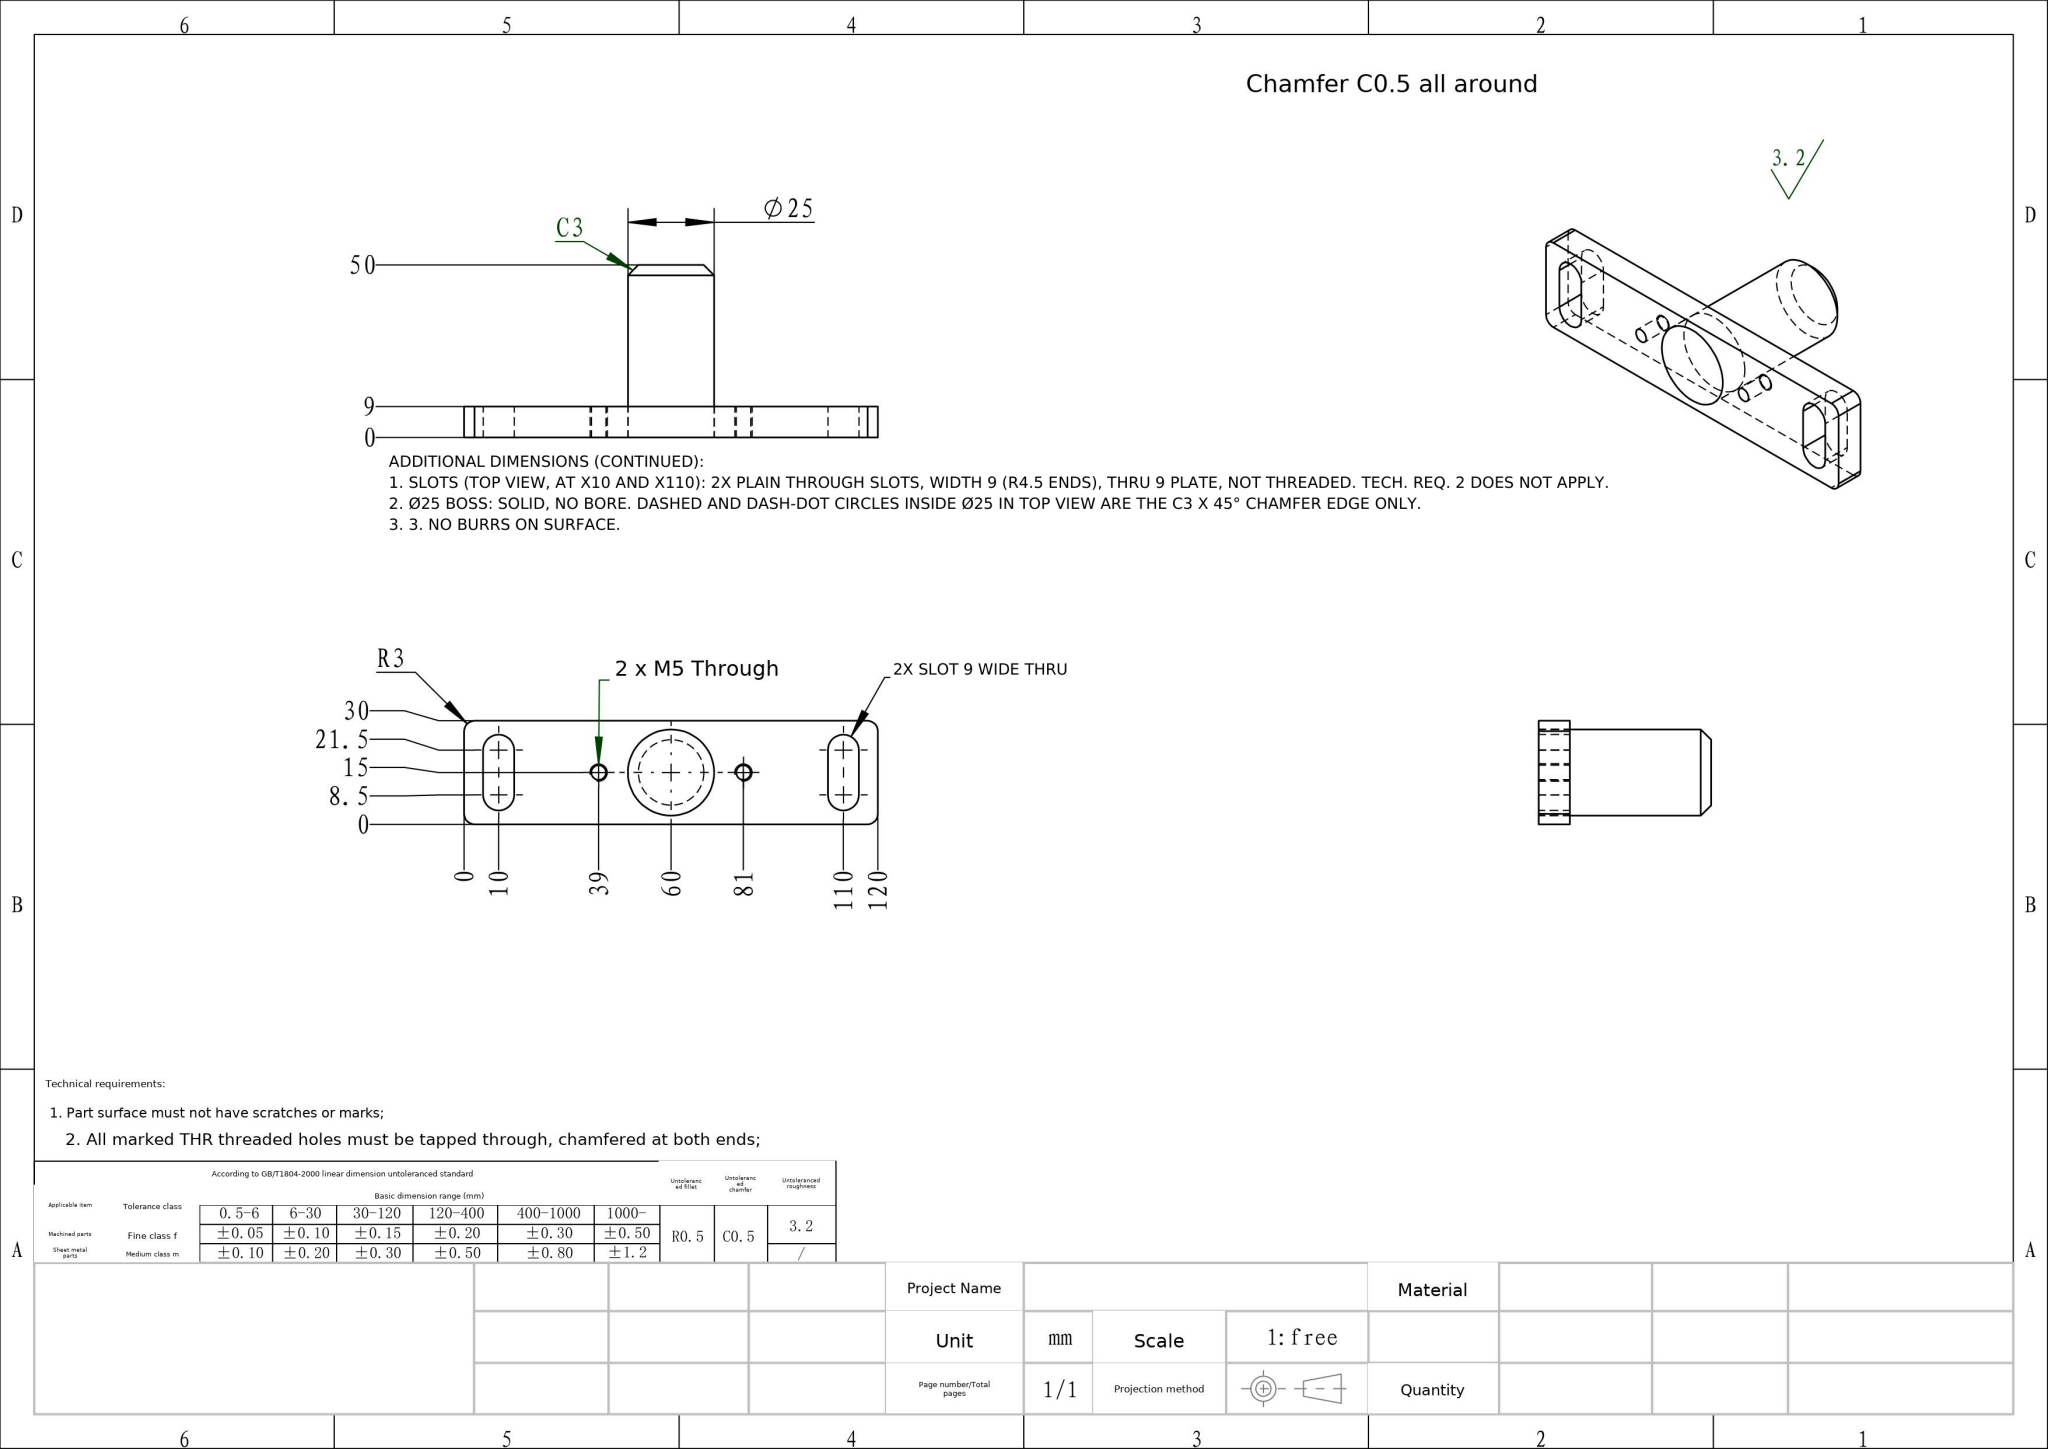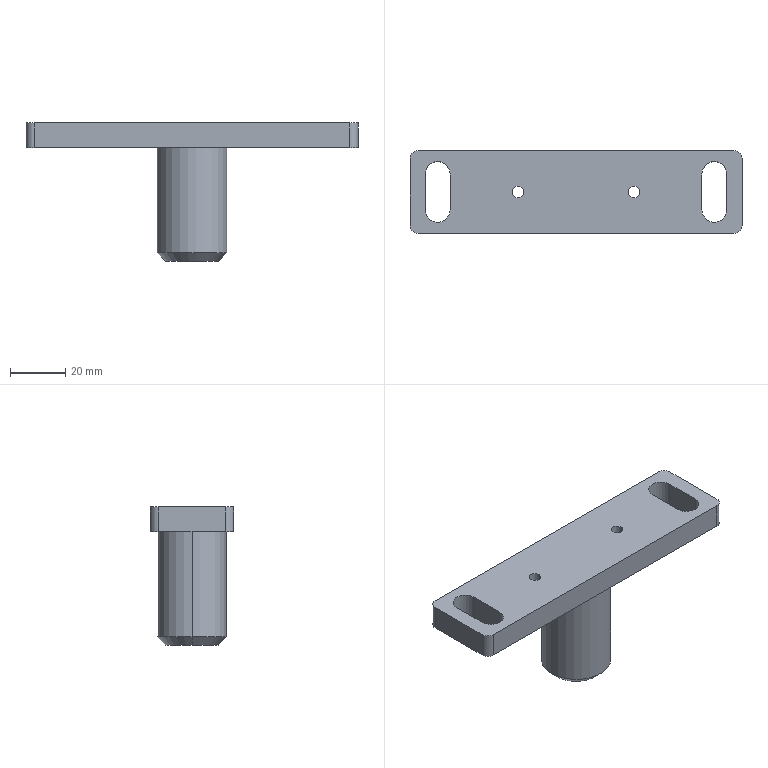Part | NX | mm | 1 solid | 27 faces | box 120 x 30 x 50 mm | volume 48631 mm3 | cylinder 14 | plane 11 | cone 2 | commonest cylinder face diameters 4.2 x4 6 x4 9 x4 25 x2
STEP:
#1=COLOUR_RGB('',0.7922,0.8196,0.9333);
#2=FILL_AREA_STYLE_COLOUR('',#1);
#3=FILL_AREA_STYLE('',(#2));
#4=SURFACE_STYLE_FILL_AREA(#3);
#5=SURFACE_SIDE_STYLE('',(#4));
#6=SURFACE_STYLE_USAGE(.BOTH.,#5);
#7=PRESENTATION_STYLE_ASSIGNMENT((#6));
#8=CARTESIAN_POINT('',(-9.5,0.,-45.5));
#9=VERTEX_POINT('',#8);
#10=CARTESIAN_POINT('',(-12.5,0.,-42.5));
#11=VERTEX_POINT('',#10);
#12=CARTESIAN_POINT('',(-12.5,0.,-42.5));
#13=DIRECTION('',(-0.7071,0.,0.7071));
#14=VECTOR('',#13,1000.);
#15=LINE('',#12,#14);
#16=EDGE_CURVE('',#9,#11,#15,.T.);
#17=ORIENTED_EDGE('',*,*,#16,.F.);
#18=CARTESIAN_POINT('',(9.5,0.,-45.5));
#19=VERTEX_POINT('',#18);
#20=CARTESIAN_POINT('',(0.,0.,-45.5));
#21=DIRECTION('',(0.,0.,-1.));
#22=DIRECTION('',(1.,0.,0.));
#23=AXIS2_PLACEMENT_3D('',#20,#21,#22);
#24=CIRCLE('',#23,9.5);
#25=EDGE_CURVE('',#19,#9,#24,.T.);
#26=ORIENTED_EDGE('',*,*,#25,.F.);
#27=CARTESIAN_POINT('',(12.5,0.,-42.5));
#28=VERTEX_POINT('',#27);
#29=CARTESIAN_POINT('',(12.5,0.,-42.5));
#30=DIRECTION('',(0.7071,0.,0.7071));
#31=VECTOR('',#30,1000.);
#32=LINE('',#29,#31);
#33=EDGE_CURVE('',#19,#28,#32,.T.);
#34=ORIENTED_EDGE('',*,*,#33,.T.);
#35=CARTESIAN_POINT('',(0.,0.,-42.5));
#36=DIRECTION('',(0.,0.,1.));
#37=DIRECTION('',(1.,0.,0.));
#38=AXIS2_PLACEMENT_3D('',#35,#36,#37);
#39=CIRCLE('',#38,12.5);
#40=EDGE_CURVE('',#11,#28,#39,.T.);
#41=ORIENTED_EDGE('',*,*,#40,.F.);
#42=EDGE_LOOP('',(#17,#26,#34,#41));
#43=FACE_OUTER_BOUND('',#42,.T.);
#44=CARTESIAN_POINT('',(0.,0.,-42.5));
#45=DIRECTION('',(0.,0.,1.));
#46=DIRECTION('',(1.,0.,0.));
#47=AXIS2_PLACEMENT_3D('',#44,#45,#46);
#48=CONICAL_SURFACE('',#47,12.5,0.7854);
#49=ADVANCED_FACE('',(#43),#48,.T.);
#50=ORIENTED_EDGE('',*,*,#25,.T.);
#51=CARTESIAN_POINT('',(0.,0.,-45.5));
#52=DIRECTION('',(0.,0.,-1.));
#53=DIRECTION('',(1.,0.,0.));
#54=AXIS2_PLACEMENT_3D('',#51,#52,#53);
#55=CIRCLE('',#54,9.5);
#56=EDGE_CURVE('',#9,#19,#55,.T.);
#57=ORIENTED_EDGE('',*,*,#56,.T.);
#58=EDGE_LOOP('',(#50,#57));
#59=FACE_OUTER_BOUND('',#58,.T.);
#60=CARTESIAN_POINT('',(0.,0.,-45.5));
#61=DIRECTION('',(0.,0.,1.));
#62=DIRECTION('',(1.,0.,0.));
#63=AXIS2_PLACEMENT_3D('',#60,#61,#62);
#64=PLANE('',#63);
#65=ADVANCED_FACE('',(#59),#64,.F.);
#66=CARTESIAN_POINT('',(-12.5,0.,-4.5));
#67=VERTEX_POINT('',#66);
#68=CARTESIAN_POINT('',(12.5,0.,-4.5));
#69=VERTEX_POINT('',#68);
#70=CARTESIAN_POINT('',(0.,0.,-4.5));
#71=DIRECTION('',(0.,0.,1.));
#72=DIRECTION('',(1.,0.,0.));
#73=AXIS2_PLACEMENT_3D('',#70,#71,#72);
#74=CIRCLE('',#73,12.5);
#75=EDGE_CURVE('',#67,#69,#74,.T.);
#76=ORIENTED_EDGE('',*,*,#75,.F.);
#77=CARTESIAN_POINT('',(-12.5,0.,-45.5));
#78=DIRECTION('',(0.,0.,1.));
#79=VECTOR('',#78,1000.);
#80=LINE('',#77,#79);
#81=EDGE_CURVE('',#11,#67,#80,.T.);
#82=ORIENTED_EDGE('',*,*,#81,.F.);
#83=ORIENTED_EDGE('',*,*,#40,.T.);
#84=CARTESIAN_POINT('',(12.5,0.,-45.5));
#85=DIRECTION('',(0.,0.,1.));
#86=VECTOR('',#85,1000.);
#87=LINE('',#84,#86);
#88=EDGE_CURVE('',#28,#69,#87,.T.);
#89=ORIENTED_EDGE('',*,*,#88,.T.);
#90=EDGE_LOOP('',(#76,#82,#83,#89));
#91=FACE_OUTER_BOUND('',#90,.T.);
#92=CARTESIAN_POINT('',(0.,0.,-45.5));
#93=DIRECTION('',(0.,0.,1.));
#94=DIRECTION('',(1.,0.,0.));
#95=AXIS2_PLACEMENT_3D('',#92,#93,#94);
#96=CYLINDRICAL_SURFACE('',#95,12.5);
#97=ADVANCED_FACE('',(#91),#96,.T.);
#98=CARTESIAN_POINT('',(0.,0.,-4.5));
#99=DIRECTION('',(0.,0.,1.));
#100=DIRECTION('',(1.,0.,0.));
#101=AXIS2_PLACEMENT_3D('',#98,#99,#100);
#102=CIRCLE('',#101,12.5);
#103=EDGE_CURVE('',#69,#67,#102,.T.);
#104=ORIENTED_EDGE('',*,*,#103,.F.);
#105=ORIENTED_EDGE('',*,*,#88,.F.);
#106=CARTESIAN_POINT('',(0.,0.,-42.5));
#107=DIRECTION('',(0.,0.,1.));
#108=DIRECTION('',(1.,0.,0.));
#109=AXIS2_PLACEMENT_3D('',#106,#107,#108);
#110=CIRCLE('',#109,12.5);
#111=EDGE_CURVE('',#28,#11,#110,.T.);
#112=ORIENTED_EDGE('',*,*,#111,.T.);
#113=ORIENTED_EDGE('',*,*,#81,.T.);
#114=EDGE_LOOP('',(#104,#105,#112,#113));
#115=FACE_OUTER_BOUND('',#114,.T.);
#116=CARTESIAN_POINT('',(0.,0.,-45.5));
#117=DIRECTION('',(0.,0.,1.));
#118=DIRECTION('',(1.,0.,0.));
#119=AXIS2_PLACEMENT_3D('',#116,#117,#118);
#120=CYLINDRICAL_SURFACE('',#119,12.5);
#121=ADVANCED_FACE('',(#115),#120,.T.);
#122=ORIENTED_EDGE('',*,*,#56,.F.);
#123=ORIENTED_EDGE('',*,*,#16,.T.);
#124=ORIENTED_EDGE('',*,*,#111,.F.);
#125=ORIENTED_EDGE('',*,*,#33,.F.);
#126=EDGE_LOOP('',(#122,#123,#124,#125));
#127=FACE_OUTER_BOUND('',#126,.T.);
#128=CARTESIAN_POINT('',(0.,0.,-42.5));
#129=DIRECTION('',(0.,0.,1.));
#130=DIRECTION('',(1.,0.,0.));
#131=AXIS2_PLACEMENT_3D('',#128,#129,#130);
#132=CONICAL_SURFACE('',#131,12.5,0.7854);
#133=ADVANCED_FACE('',(#127),#132,.T.);
#134=CARTESIAN_POINT('',(23.1,-0.,4.5));
#135=VERTEX_POINT('',#134);
#136=CARTESIAN_POINT('',(23.1,-0.,-4.5));
#137=VERTEX_POINT('',#136);
#138=CARTESIAN_POINT('',(23.1,-0.,-4.5));
#139=DIRECTION('',(0.,0.,-1.));
#140=VECTOR('',#139,1000.);
#141=LINE('',#138,#140);
#142=EDGE_CURVE('',#135,#137,#141,.T.);
#143=ORIENTED_EDGE('',*,*,#142,.F.);
#144=CARTESIAN_POINT('',(18.9,-0.,4.5));
#145=VERTEX_POINT('',#144);
#146=CARTESIAN_POINT('',(21.,-0.,4.5));
#147=DIRECTION('',(0.,0.,-1.));
#148=DIRECTION('',(-1.,0.,0.));
#149=AXIS2_PLACEMENT_3D('',#146,#147,#148);
#150=CIRCLE('',#149,2.1);
#151=EDGE_CURVE('',#145,#135,#150,.T.);
#152=ORIENTED_EDGE('',*,*,#151,.F.);
#153=CARTESIAN_POINT('',(18.9,-0.,-4.5));
#154=VERTEX_POINT('',#153);
#155=CARTESIAN_POINT('',(18.9,-0.,-4.5));
#156=DIRECTION('',(0.,0.,-1.));
#157=VECTOR('',#156,1000.);
#158=LINE('',#155,#157);
#159=EDGE_CURVE('',#145,#154,#158,.T.);
#160=ORIENTED_EDGE('',*,*,#159,.T.);
#161=CARTESIAN_POINT('',(21.,-0.,-4.5));
#162=DIRECTION('',(0.,0.,-1.));
#163=DIRECTION('',(-1.,0.,0.));
#164=AXIS2_PLACEMENT_3D('',#161,#162,#163);
#165=CIRCLE('',#164,2.1);
#166=EDGE_CURVE('',#154,#137,#165,.T.);
#167=ORIENTED_EDGE('',*,*,#166,.T.);
#168=EDGE_LOOP('',(#143,#152,#160,#167));
#169=FACE_OUTER_BOUND('',#168,.T.);
#170=CARTESIAN_POINT('',(21.,-0.,-4.5));
#171=DIRECTION('',(0.,0.,-1.));
#172=DIRECTION('',(-1.,0.,0.));
#173=AXIS2_PLACEMENT_3D('',#170,#171,#172);
#174=CYLINDRICAL_SURFACE('',#173,2.1);
#175=ADVANCED_FACE('',(#169),#174,.F.);
#176=CARTESIAN_POINT('',(-18.9,0.,4.5));
#177=VERTEX_POINT('',#176);
#178=CARTESIAN_POINT('',(-18.9,0.,-4.5));
#179=VERTEX_POINT('',#178);
#180=CARTESIAN_POINT('',(-18.9,0.,-4.5));
#181=DIRECTION('',(0.,0.,-1.));
#182=VECTOR('',#181,1000.);
#183=LINE('',#180,#182);
#184=EDGE_CURVE('',#177,#179,#183,.T.);
#185=ORIENTED_EDGE('',*,*,#184,.F.);
#186=CARTESIAN_POINT('',(-23.1,0.,4.5));
#187=VERTEX_POINT('',#186);
#188=CARTESIAN_POINT('',(-21.,0.,4.5));
#189=DIRECTION('',(0.,0.,-1.));
#190=DIRECTION('',(-1.,0.,0.));
#191=AXIS2_PLACEMENT_3D('',#188,#189,#190);
#192=CIRCLE('',#191,2.1);
#193=EDGE_CURVE('',#187,#177,#192,.T.);
#194=ORIENTED_EDGE('',*,*,#193,.F.);
#195=CARTESIAN_POINT('',(-23.1,0.,-4.5));
#196=VERTEX_POINT('',#195);
#197=CARTESIAN_POINT('',(-23.1,0.,-4.5));
#198=DIRECTION('',(0.,0.,-1.));
#199=VECTOR('',#198,1000.);
#200=LINE('',#197,#199);
#201=EDGE_CURVE('',#187,#196,#200,.T.);
#202=ORIENTED_EDGE('',*,*,#201,.T.);
#203=CARTESIAN_POINT('',(-21.,0.,-4.5));
#204=DIRECTION('',(0.,0.,-1.));
#205=DIRECTION('',(-1.,0.,0.));
#206=AXIS2_PLACEMENT_3D('',#203,#204,#205);
#207=CIRCLE('',#206,2.1);
#208=EDGE_CURVE('',#196,#179,#207,.T.);
#209=ORIENTED_EDGE('',*,*,#208,.T.);
#210=EDGE_LOOP('',(#185,#194,#202,#209));
#211=FACE_OUTER_BOUND('',#210,.T.);
#212=CARTESIAN_POINT('',(-21.,0.,-4.5));
#213=DIRECTION('',(0.,0.,-1.));
#214=DIRECTION('',(-1.,0.,0.));
#215=AXIS2_PLACEMENT_3D('',#212,#213,#214);
#216=CYLINDRICAL_SURFACE('',#215,2.1);
#217=ADVANCED_FACE('',(#211),#216,.F.);
#218=CARTESIAN_POINT('',(60.,12.,4.5));
#219=VERTEX_POINT('',#218);
#220=CARTESIAN_POINT('',(57.,15.,4.5));
#221=VERTEX_POINT('',#220);
#222=CARTESIAN_POINT('',(57.,12.,4.5));
#223=DIRECTION('',(0.,0.,1.));
#224=DIRECTION('',(-1.,0.,0.));
#225=AXIS2_PLACEMENT_3D('',#222,#223,#224);
#226=CIRCLE('',#225,3.);
#227=EDGE_CURVE('',#219,#221,#226,.T.);
#228=ORIENTED_EDGE('',*,*,#227,.F.);
#229=CARTESIAN_POINT('',(60.,12.,-4.5));
#230=VERTEX_POINT('',#229);
#231=CARTESIAN_POINT('',(60.,12.,4.5));
#232=DIRECTION('',(0.,0.,1.));
#233=VECTOR('',#232,1000.);
#234=LINE('',#231,#233);
#235=EDGE_CURVE('',#230,#219,#234,.T.);
#236=ORIENTED_EDGE('',*,*,#235,.F.);
#237=CARTESIAN_POINT('',(57.,15.,-4.5));
#238=VERTEX_POINT('',#237);
#239=CARTESIAN_POINT('',(57.,12.,-4.5));
#240=DIRECTION('',(0.,0.,-1.));
#241=DIRECTION('',(-1.,0.,0.));
#242=AXIS2_PLACEMENT_3D('',#239,#240,#241);
#243=CIRCLE('',#242,3.);
#244=EDGE_CURVE('',#238,#230,#243,.T.);
#245=ORIENTED_EDGE('',*,*,#244,.F.);
#246=CARTESIAN_POINT('',(57.,15.,4.5));
#247=DIRECTION('',(0.,0.,-1.));
#248=VECTOR('',#247,1000.);
#249=LINE('',#246,#248);
#250=EDGE_CURVE('',#221,#238,#249,.T.);
#251=ORIENTED_EDGE('',*,*,#250,.F.);
#252=EDGE_LOOP('',(#228,#236,#245,#251));
#253=FACE_OUTER_BOUND('',#252,.T.);
#254=CARTESIAN_POINT('',(57.,12.,4.5));
#255=DIRECTION('',(0.,0.,-1.));
#256=DIRECTION('',(-1.,0.,0.));
#257=AXIS2_PLACEMENT_3D('',#254,#255,#256);
#258=CYLINDRICAL_SURFACE('',#257,3.);
#259=ADVANCED_FACE('',(#253),#258,.T.);
#260=CARTESIAN_POINT('',(57.,-15.,4.5));
#261=VERTEX_POINT('',#260);
#262=CARTESIAN_POINT('',(60.,-12.,4.5));
#263=VERTEX_POINT('',#262);
#264=CARTESIAN_POINT('',(57.,-12.,4.5));
#265=DIRECTION('',(0.,0.,1.));
#266=DIRECTION('',(-1.,0.,0.));
#267=AXIS2_PLACEMENT_3D('',#264,#265,#266);
#268=CIRCLE('',#267,3.);
#269=EDGE_CURVE('',#261,#263,#268,.T.);
#270=ORIENTED_EDGE('',*,*,#269,.F.);
#271=CARTESIAN_POINT('',(57.,-15.,-4.5));
#272=VERTEX_POINT('',#271);
#273=CARTESIAN_POINT('',(57.,-15.,4.5));
#274=DIRECTION('',(0.,0.,1.));
#275=VECTOR('',#274,1000.);
#276=LINE('',#273,#275);
#277=EDGE_CURVE('',#272,#261,#276,.T.);
#278=ORIENTED_EDGE('',*,*,#277,.F.);
#279=CARTESIAN_POINT('',(60.,-12.,-4.5));
#280=VERTEX_POINT('',#279);
#281=CARTESIAN_POINT('',(57.,-12.,-4.5));
#282=DIRECTION('',(0.,0.,-1.));
#283=DIRECTION('',(-1.,0.,0.));
#284=AXIS2_PLACEMENT_3D('',#281,#282,#283);
#285=CIRCLE('',#284,3.);
#286=EDGE_CURVE('',#280,#272,#285,.T.);
#287=ORIENTED_EDGE('',*,*,#286,.F.);
#288=CARTESIAN_POINT('',(60.,-12.,4.5));
#289=DIRECTION('',(0.,0.,-1.));
#290=VECTOR('',#289,1000.);
#291=LINE('',#288,#290);
#292=EDGE_CURVE('',#263,#280,#291,.T.);
#293=ORIENTED_EDGE('',*,*,#292,.F.);
#294=EDGE_LOOP('',(#270,#278,#287,#293));
#295=FACE_OUTER_BOUND('',#294,.T.);
#296=CARTESIAN_POINT('',(57.,-12.,4.5));
#297=DIRECTION('',(0.,0.,-1.));
#298=DIRECTION('',(-1.,0.,0.));
#299=AXIS2_PLACEMENT_3D('',#296,#297,#298);
#300=CYLINDRICAL_SURFACE('',#299,3.);
#301=ADVANCED_FACE('',(#295),#300,.T.);
#302=CARTESIAN_POINT('',(-57.,15.,4.5));
#303=VERTEX_POINT('',#302);
#304=CARTESIAN_POINT('',(-60.,12.,4.5));
#305=VERTEX_POINT('',#304);
#306=CARTESIAN_POINT('',(-57.,12.,4.5));
#307=DIRECTION('',(0.,0.,1.));
#308=DIRECTION('',(-1.,0.,0.));
#309=AXIS2_PLACEMENT_3D('',#306,#307,#308);
#310=CIRCLE('',#309,3.);
#311=EDGE_CURVE('',#303,#305,#310,.T.);
#312=ORIENTED_EDGE('',*,*,#311,.F.);
#313=CARTESIAN_POINT('',(-57.,15.,-4.5));
#314=VERTEX_POINT('',#313);
#315=CARTESIAN_POINT('',(-57.,15.,4.5));
#316=DIRECTION('',(0.,0.,1.));
#317=VECTOR('',#316,1000.);
#318=LINE('',#315,#317);
#319=EDGE_CURVE('',#314,#303,#318,.T.);
#320=ORIENTED_EDGE('',*,*,#319,.F.);
#321=CARTESIAN_POINT('',(-60.,12.,-4.5));
#322=VERTEX_POINT('',#321);
#323=CARTESIAN_POINT('',(-57.,12.,-4.5));
#324=DIRECTION('',(0.,0.,-1.));
#325=DIRECTION('',(-1.,0.,0.));
#326=AXIS2_PLACEMENT_3D('',#323,#324,#325);
#327=CIRCLE('',#326,3.);
#328=EDGE_CURVE('',#322,#314,#327,.T.);
#329=ORIENTED_EDGE('',*,*,#328,.F.);
#330=CARTESIAN_POINT('',(-60.,12.,4.5));
#331=DIRECTION('',(0.,0.,-1.));
#332=VECTOR('',#331,1000.);
#333=LINE('',#330,#332);
#334=EDGE_CURVE('',#305,#322,#333,.T.);
#335=ORIENTED_EDGE('',*,*,#334,.F.);
#336=EDGE_LOOP('',(#312,#320,#329,#335));
#337=FACE_OUTER_BOUND('',#336,.T.);
#338=CARTESIAN_POINT('',(-57.,12.,4.5));
#339=DIRECTION('',(0.,0.,-1.));
#340=DIRECTION('',(-1.,0.,0.));
#341=AXIS2_PLACEMENT_3D('',#338,#339,#340);
#342=CYLINDRICAL_SURFACE('',#341,3.);
#343=ADVANCED_FACE('',(#337),#342,.T.);
#344=CARTESIAN_POINT('',(-60.,-12.,4.5));
#345=VERTEX_POINT('',#344);
#346=CARTESIAN_POINT('',(-57.,-15.,4.5));
#347=VERTEX_POINT('',#346);
#348=CARTESIAN_POINT('',(-57.,-12.,4.5));
#349=DIRECTION('',(0.,0.,1.));
#350=DIRECTION('',(-1.,0.,0.));
#351=AXIS2_PLACEMENT_3D('',#348,#349,#350);
#352=CIRCLE('',#351,3.);
#353=EDGE_CURVE('',#345,#347,#352,.T.);
#354=ORIENTED_EDGE('',*,*,#353,.F.);
#355=CARTESIAN_POINT('',(-60.,-12.,-4.5));
#356=VERTEX_POINT('',#355);
#357=CARTESIAN_POINT('',(-60.,-12.,4.5));
#358=DIRECTION('',(0.,0.,1.));
#359=VECTOR('',#358,1000.);
#360=LINE('',#357,#359);
#361=EDGE_CURVE('',#356,#345,#360,.T.);
#362=ORIENTED_EDGE('',*,*,#361,.F.);
#363=CARTESIAN_POINT('',(-57.,-15.,-4.5));
#364=VERTEX_POINT('',#363);
#365=CARTESIAN_POINT('',(-57.,-12.,-4.5));
#366=DIRECTION('',(0.,0.,-1.));
#367=DIRECTION('',(-1.,0.,0.));
#368=AXIS2_PLACEMENT_3D('',#365,#366,#367);
#369=CIRCLE('',#368,3.);
#370=EDGE_CURVE('',#364,#356,#369,.T.);
#371=ORIENTED_EDGE('',*,*,#370,.F.);
#372=CARTESIAN_POINT('',(-57.,-15.,4.5));
#373=DIRECTION('',(0.,0.,-1.));
#374=VECTOR('',#373,1000.);
#375=LINE('',#372,#374);
#376=EDGE_CURVE('',#347,#364,#375,.T.);
#377=ORIENTED_EDGE('',*,*,#376,.F.);
#378=EDGE_LOOP('',(#354,#362,#371,#377));
#379=FACE_OUTER_BOUND('',#378,.T.);
#380=CARTESIAN_POINT('',(-57.,-12.,4.5));
#381=DIRECTION('',(0.,0.,-1.));
#382=DIRECTION('',(-1.,0.,0.));
#383=AXIS2_PLACEMENT_3D('',#380,#381,#382);
#384=CYLINDRICAL_SURFACE('',#383,3.);
#385=ADVANCED_FACE('',(#379),#384,.T.);
#386=CARTESIAN_POINT('',(54.5,-6.5,4.5));
#387=VERTEX_POINT('',#386);
#388=CARTESIAN_POINT('',(54.5,6.5,4.5));
#389=VERTEX_POINT('',#388);
#390=CARTESIAN_POINT('',(54.5,-6.5,4.5));
#391=DIRECTION('',(0.,1.,0.));
#392=VECTOR('',#391,1000.);
#393=LINE('',#390,#392);
#394=EDGE_CURVE('',#387,#389,#393,.T.);
#395=ORIENTED_EDGE('',*,*,#394,.T.);
#396=CARTESIAN_POINT('',(54.5,6.5,-4.5));
#397=VERTEX_POINT('',#396);
#398=CARTESIAN_POINT('',(54.5,6.5,-4.5));
#399=DIRECTION('',(0.,0.,1.));
#400=VECTOR('',#399,1000.);
#401=LINE('',#398,#400);
#402=EDGE_CURVE('',#397,#389,#401,.T.);
#403=ORIENTED_EDGE('',*,*,#402,.F.);
#404=CARTESIAN_POINT('',(54.5,-6.5,-4.5));
#405=VERTEX_POINT('',#404);
#406=CARTESIAN_POINT('',(54.5,-6.5,-4.5));
#407=DIRECTION('',(0.,1.,0.));
#408=VECTOR('',#407,1000.);
#409=LINE('',#406,#408);
#410=EDGE_CURVE('',#405,#397,#409,.T.);
#411=ORIENTED_EDGE('',*,*,#410,.F.);
#412=CARTESIAN_POINT('',(54.5,-6.5,-4.5));
#413=DIRECTION('',(0.,0.,1.));
#414=VECTOR('',#413,1000.);
#415=LINE('',#412,#414);
#416=EDGE_CURVE('',#405,#387,#415,.T.);
#417=ORIENTED_EDGE('',*,*,#416,.T.);
#418=EDGE_LOOP('',(#395,#403,#411,#417));
#419=FACE_OUTER_BOUND('',#418,.T.);
#420=CARTESIAN_POINT('',(54.5,-6.5,-4.5));
#421=DIRECTION('',(1.,0.,0.));
#422=DIRECTION('',(0.,1.,0.));
#423=AXIS2_PLACEMENT_3D('',#420,#421,#422);
#424=PLANE('',#423);
#425=ADVANCED_FACE('',(#419),#424,.F.);
#426=CARTESIAN_POINT('',(45.5,6.5,4.5));
#427=VERTEX_POINT('',#426);
#428=CARTESIAN_POINT('',(50.,6.5,4.5));
#429=DIRECTION('',(0.,0.,1.));
#430=DIRECTION('',(-1.,0.,0.));
#431=AXIS2_PLACEMENT_3D('',#428,#429,#430);
#432=CIRCLE('',#431,4.5);
#433=EDGE_CURVE('',#389,#427,#432,.T.);
#434=ORIENTED_EDGE('',*,*,#433,.T.);
#435=CARTESIAN_POINT('',(45.5,6.5,-4.5));
#436=VERTEX_POINT('',#435);
#437=CARTESIAN_POINT('',(45.5,6.5,-4.5));
#438=DIRECTION('',(0.,0.,1.));
#439=VECTOR('',#438,1000.);
#440=LINE('',#437,#439);
#441=EDGE_CURVE('',#436,#427,#440,.T.);
#442=ORIENTED_EDGE('',*,*,#441,.F.);
#443=CARTESIAN_POINT('',(50.,6.5,-4.5));
#444=DIRECTION('',(0.,0.,1.));
#445=DIRECTION('',(-1.,0.,0.));
#446=AXIS2_PLACEMENT_3D('',#443,#444,#445);
#447=CIRCLE('',#446,4.5);
#448=EDGE_CURVE('',#397,#436,#447,.T.);
#449=ORIENTED_EDGE('',*,*,#448,.F.);
#450=ORIENTED_EDGE('',*,*,#402,.T.);
#451=EDGE_LOOP('',(#434,#442,#449,#450));
#452=FACE_OUTER_BOUND('',#451,.T.);
#453=CARTESIAN_POINT('',(50.,6.5,-4.5));
#454=DIRECTION('',(0.,0.,1.));
#455=DIRECTION('',(1.,0.,0.));
#456=AXIS2_PLACEMENT_3D('',#453,#454,#455);
#457=CYLINDRICAL_SURFACE('',#456,4.5);
#458=ADVANCED_FACE('',(#452),#457,.F.);
#459=CARTESIAN_POINT('',(45.5,-6.5,4.5));
#460=VERTEX_POINT('',#459);
#461=CARTESIAN_POINT('',(45.5,-6.5,4.5));
#462=DIRECTION('',(0.,-1.,0.));
#463=VECTOR('',#462,1000.);
#464=LINE('',#461,#463);
#465=EDGE_CURVE('',#427,#460,#464,.T.);
#466=ORIENTED_EDGE('',*,*,#465,.T.);
#467=CARTESIAN_POINT('',(45.5,-6.5,-4.5));
#468=VERTEX_POINT('',#467);
#469=CARTESIAN_POINT('',(45.5,-6.5,-4.5));
#470=DIRECTION('',(0.,0.,1.));
#471=VECTOR('',#470,1000.);
#472=LINE('',#469,#471);
#473=EDGE_CURVE('',#468,#460,#472,.T.);
#474=ORIENTED_EDGE('',*,*,#473,.F.);
#475=CARTESIAN_POINT('',(45.5,-6.5,-4.5));
#476=DIRECTION('',(0.,-1.,0.));
#477=VECTOR('',#476,1000.);
#478=LINE('',#475,#477);
#479=EDGE_CURVE('',#436,#468,#478,.T.);
#480=ORIENTED_EDGE('',*,*,#479,.F.);
#481=ORIENTED_EDGE('',*,*,#441,.T.);
#482=EDGE_LOOP('',(#466,#474,#480,#481));
#483=FACE_OUTER_BOUND('',#482,.T.);
#484=CARTESIAN_POINT('',(45.5,-6.5,-4.5));
#485=DIRECTION('',(-1.,0.,0.));
#486=DIRECTION('',(0.,0.,1.));
#487=AXIS2_PLACEMENT_3D('',#484,#485,#486);
#488=PLANE('',#487);
#489=ADVANCED_FACE('',(#483),#488,.F.);
#490=CARTESIAN_POINT('',(50.,-6.5,4.5));
#491=DIRECTION('',(0.,0.,1.));
#492=DIRECTION('',(-1.,0.,0.));
#493=AXIS2_PLACEMENT_3D('',#490,#491,#492);
#494=CIRCLE('',#493,4.5);
#495=EDGE_CURVE('',#460,#387,#494,.T.);
#496=ORIENTED_EDGE('',*,*,#495,.T.);
#497=ORIENTED_EDGE('',*,*,#416,.F.);
#498=CARTESIAN_POINT('',(50.,-6.5,-4.5));
#499=DIRECTION('',(0.,0.,1.));
#500=DIRECTION('',(-1.,0.,0.));
#501=AXIS2_PLACEMENT_3D('',#498,#499,#500);
#502=CIRCLE('',#501,4.5);
#503=EDGE_CURVE('',#468,#405,#502,.T.);
#504=ORIENTED_EDGE('',*,*,#503,.F.);
#505=ORIENTED_EDGE('',*,*,#473,.T.);
#506=EDGE_LOOP('',(#496,#497,#504,#505));
#507=FACE_OUTER_BOUND('',#506,.T.);
#508=CARTESIAN_POINT('',(50.,-6.5,-4.5));
#509=DIRECTION('',(0.,0.,1.));
#510=DIRECTION('',(1.,0.,0.));
#511=AXIS2_PLACEMENT_3D('',#508,#509,#510);
#512=CYLINDRICAL_SURFACE('',#511,4.5);
#513=ADVANCED_FACE('',(#507),#512,.F.);
#514=CARTESIAN_POINT('',(-45.5,-6.5,4.5));
#515=VERTEX_POINT('',#514);
#516=CARTESIAN_POINT('',(-45.5,6.5,4.5));
#517=VERTEX_POINT('',#516);
#518=CARTESIAN_POINT('',(-45.5,-6.5,4.5));
#519=DIRECTION('',(0.,1.,0.));
#520=VECTOR('',#519,1000.);
#521=LINE('',#518,#520);
#522=EDGE_CURVE('',#515,#517,#521,.T.);
#523=ORIENTED_EDGE('',*,*,#522,.T.);
#524=CARTESIAN_POINT('',(-45.5,6.5,-4.5));
#525=VERTEX_POINT('',#524);
#526=CARTESIAN_POINT('',(-45.5,6.5,-4.5));
#527=DIRECTION('',(0.,0.,1.));
#528=VECTOR('',#527,1000.);
#529=LINE('',#526,#528);
#530=EDGE_CURVE('',#525,#517,#529,.T.);
#531=ORIENTED_EDGE('',*,*,#530,.F.);
#532=CARTESIAN_POINT('',(-45.5,-6.5,-4.5));
#533=VERTEX_POINT('',#532);
#534=CARTESIAN_POINT('',(-45.5,-6.5,-4.5));
#535=DIRECTION('',(0.,1.,0.));
#536=VECTOR('',#535,1000.);
#537=LINE('',#534,#536);
#538=EDGE_CURVE('',#533,#525,#537,.T.);
#539=ORIENTED_EDGE('',*,*,#538,.F.);
#540=CARTESIAN_POINT('',(-45.5,-6.5,-4.5));
#541=DIRECTION('',(0.,0.,1.));
#542=VECTOR('',#541,1000.);
#543=LINE('',#540,#542);
#544=EDGE_CURVE('',#533,#515,#543,.T.);
#545=ORIENTED_EDGE('',*,*,#544,.T.);
#546=EDGE_LOOP('',(#523,#531,#539,#545));
#547=FACE_OUTER_BOUND('',#546,.T.);
#548=CARTESIAN_POINT('',(-45.5,-6.5,-4.5));
#549=DIRECTION('',(1.,0.,0.));
#550=DIRECTION('',(0.,1.,0.));
#551=AXIS2_PLACEMENT_3D('',#548,#549,#550);
#552=PLANE('',#551);
#553=ADVANCED_FACE('',(#547),#552,.F.);
#554=CARTESIAN_POINT('',(-54.5,6.5,4.5));
#555=VERTEX_POINT('',#554);
#556=CARTESIAN_POINT('',(-50.,6.5,4.5));
#557=DIRECTION('',(0.,0.,1.));
#558=DIRECTION('',(1.,0.,0.));
#559=AXIS2_PLACEMENT_3D('',#556,#557,#558);
#560=CIRCLE('',#559,4.5);
#561=EDGE_CURVE('',#517,#555,#560,.T.);
#562=ORIENTED_EDGE('',*,*,#561,.T.);
#563=CARTESIAN_POINT('',(-54.5,6.5,-4.5));
#564=VERTEX_POINT('',#563);
#565=CARTESIAN_POINT('',(-54.5,6.5,-4.5));
#566=DIRECTION('',(0.,0.,1.));
#567=VECTOR('',#566,1000.);
#568=LINE('',#565,#567);
#569=EDGE_CURVE('',#564,#555,#568,.T.);
#570=ORIENTED_EDGE('',*,*,#569,.F.);
#571=CARTESIAN_POINT('',(-50.,6.5,-4.5));
#572=DIRECTION('',(0.,0.,1.));
#573=DIRECTION('',(1.,0.,0.));
#574=AXIS2_PLACEMENT_3D('',#571,#572,#573);
#575=CIRCLE('',#574,4.5);
#576=EDGE_CURVE('',#525,#564,#575,.T.);
#577=ORIENTED_EDGE('',*,*,#576,.F.);
#578=ORIENTED_EDGE('',*,*,#530,.T.);
#579=EDGE_LOOP('',(#562,#570,#577,#578));
#580=FACE_OUTER_BOUND('',#579,.T.);
#581=CARTESIAN_POINT('',(-50.,6.5,-4.5));
#582=DIRECTION('',(0.,0.,1.));
#583=DIRECTION('',(1.,0.,0.));
#584=AXIS2_PLACEMENT_3D('',#581,#582,#583);
#585=CYLINDRICAL_SURFACE('',#584,4.5);
#586=ADVANCED_FACE('',(#580),#585,.F.);
#587=CARTESIAN_POINT('',(-54.5,-6.5,4.5));
#588=VERTEX_POINT('',#587);
#589=CARTESIAN_POINT('',(-54.5,-6.5,4.5));
#590=DIRECTION('',(0.,-1.,0.));
#591=VECTOR('',#590,1000.);
#592=LINE('',#589,#591);
#593=EDGE_CURVE('',#555,#588,#592,.T.);
#594=ORIENTED_EDGE('',*,*,#593,.T.);
#595=CARTESIAN_POINT('',(-54.5,-6.5,-4.5));
#596=VERTEX_POINT('',#595);
#597=CARTESIAN_POINT('',(-54.5,-6.5,-4.5));
#598=DIRECTION('',(0.,0.,1.));
#599=VECTOR('',#598,1000.);
#600=LINE('',#597,#599);
#601=EDGE_CURVE('',#596,#588,#600,.T.);
#602=ORIENTED_EDGE('',*,*,#601,.F.);
#603=CARTESIAN_POINT('',(-54.5,-6.5,-4.5));
#604=DIRECTION('',(0.,-1.,0.));
#605=VECTOR('',#604,1000.);
#606=LINE('',#603,#605);
#607=EDGE_CURVE('',#564,#596,#606,.T.);
#608=ORIENTED_EDGE('',*,*,#607,.F.);
#609=ORIENTED_EDGE('',*,*,#569,.T.);
#610=EDGE_LOOP('',(#594,#602,#608,#609));
#611=FACE_OUTER_BOUND('',#610,.T.);
#612=CARTESIAN_POINT('',(-54.5,-6.5,-4.5));
#613=DIRECTION('',(-1.,0.,0.));
#614=DIRECTION('',(0.,0.,1.));
#615=AXIS2_PLACEMENT_3D('',#612,#613,#614);
#616=PLANE('',#615);
#617=ADVANCED_FACE('',(#611),#616,.F.);
#618=CARTESIAN_POINT('',(-50.,-6.5,4.5));
#619=DIRECTION('',(0.,0.,1.));
#620=DIRECTION('',(1.,0.,0.));
#621=AXIS2_PLACEMENT_3D('',#618,#619,#620);
#622=CIRCLE('',#621,4.5);
#623=EDGE_CURVE('',#588,#515,#622,.T.);
#624=ORIENTED_EDGE('',*,*,#623,.T.);
#625=ORIENTED_EDGE('',*,*,#544,.F.);
#626=CARTESIAN_POINT('',(-50.,-6.5,-4.5));
#627=DIRECTION('',(0.,0.,1.));
#628=DIRECTION('',(1.,0.,0.));
#629=AXIS2_PLACEMENT_3D('',#626,#627,#628);
#630=CIRCLE('',#629,4.5);
#631=EDGE_CURVE('',#596,#533,#630,.T.);
#632=ORIENTED_EDGE('',*,*,#631,.F.);
#633=ORIENTED_EDGE('',*,*,#601,.T.);
#634=EDGE_LOOP('',(#624,#625,#632,#633));
#635=FACE_OUTER_BOUND('',#634,.T.);
#636=CARTESIAN_POINT('',(-50.,-6.5,-4.5));
#637=DIRECTION('',(0.,0.,1.));
#638=DIRECTION('',(1.,0.,0.));
#639=AXIS2_PLACEMENT_3D('',#636,#637,#638);
#640=CYLINDRICAL_SURFACE('',#639,4.5);
#641=ADVANCED_FACE('',(#635),#640,.F.);
#642=ORIENTED_EDGE('',*,*,#631,.T.);
#643=ORIENTED_EDGE('',*,*,#538,.T.);
#644=ORIENTED_EDGE('',*,*,#576,.T.);
#645=ORIENTED_EDGE('',*,*,#607,.T.);
#646=EDGE_LOOP('',(#642,#643,#644,#645));
#647=FACE_BOUND('',#646,.T.);
#648=ORIENTED_EDGE('',*,*,#103,.T.);
#649=ORIENTED_EDGE('',*,*,#75,.T.);
#650=EDGE_LOOP('',(#648,#649));
#651=FACE_BOUND('',#650,.T.);
#652=ORIENTED_EDGE('',*,*,#503,.T.);
#653=ORIENTED_EDGE('',*,*,#410,.T.);
#654=ORIENTED_EDGE('',*,*,#448,.T.);
#655=ORIENTED_EDGE('',*,*,#479,.T.);
#656=EDGE_LOOP('',(#652,#653,#654,#655));
#657=FACE_BOUND('',#656,.T.);
#658=ORIENTED_EDGE('',*,*,#208,.F.);
#659=CARTESIAN_POINT('',(-21.,0.,-4.5));
#660=DIRECTION('',(0.,0.,-1.));
#661=DIRECTION('',(-1.,0.,0.));
#662=AXIS2_PLACEMENT_3D('',#659,#660,#661);
#663=CIRCLE('',#662,2.1);
#664=EDGE_CURVE('',#179,#196,#663,.T.);
#665=ORIENTED_EDGE('',*,*,#664,.F.);
#666=EDGE_LOOP('',(#658,#665));
#667=FACE_BOUND('',#666,.T.);
#668=ORIENTED_EDGE('',*,*,#166,.F.);
#669=CARTESIAN_POINT('',(21.,-0.,-4.5));
#670=DIRECTION('',(0.,0.,-1.));
#671=DIRECTION('',(-1.,0.,0.));
#672=AXIS2_PLACEMENT_3D('',#669,#670,#671);
#673=CIRCLE('',#672,2.1);
#674=EDGE_CURVE('',#137,#154,#673,.T.);
#675=ORIENTED_EDGE('',*,*,#674,.F.);
#676=EDGE_LOOP('',(#668,#675));
#677=FACE_BOUND('',#676,.T.);
#678=CARTESIAN_POINT('',(-60.,-15.,-4.5));
#679=DIRECTION('',(1.,0.,0.));
#680=VECTOR('',#679,1000.);
#681=LINE('',#678,#680);
#682=EDGE_CURVE('',#364,#272,#681,.T.);
#683=ORIENTED_EDGE('',*,*,#682,.F.);
#684=ORIENTED_EDGE('',*,*,#370,.T.);
#685=CARTESIAN_POINT('',(-60.,-15.,-4.5));
#686=DIRECTION('',(0.,-1.,0.));
#687=VECTOR('',#686,1000.);
#688=LINE('',#685,#687);
#689=EDGE_CURVE('',#322,#356,#688,.T.);
#690=ORIENTED_EDGE('',*,*,#689,.F.);
#691=ORIENTED_EDGE('',*,*,#328,.T.);
#692=CARTESIAN_POINT('',(-60.,15.,-4.5));
#693=DIRECTION('',(-1.,0.,0.));
#694=VECTOR('',#693,1000.);
#695=LINE('',#692,#694);
#696=EDGE_CURVE('',#238,#314,#695,.T.);
#697=ORIENTED_EDGE('',*,*,#696,.F.);
#698=ORIENTED_EDGE('',*,*,#244,.T.);
#699=CARTESIAN_POINT('',(60.,-15.,-4.5));
#700=DIRECTION('',(0.,1.,0.));
#701=VECTOR('',#700,1000.);
#702=LINE('',#699,#701);
#703=EDGE_CURVE('',#280,#230,#702,.T.);
#704=ORIENTED_EDGE('',*,*,#703,.F.);
#705=ORIENTED_EDGE('',*,*,#286,.T.);
#706=EDGE_LOOP('',(#683,#684,#690,#691,#697,#698,#704,#705));
#707=FACE_OUTER_BOUND('',#706,.T.);
#708=CARTESIAN_POINT('',(0.,0.,-4.5));
#709=DIRECTION('',(0.,0.,-1.));
#710=DIRECTION('',(0.,-1.,0.));
#711=AXIS2_PLACEMENT_3D('',#708,#709,#710);
#712=PLANE('',#711);
#713=ADVANCED_FACE('',(#647,#651,#657,#667,#677,#707),#712,.T.);
#714=CARTESIAN_POINT('',(-60.,-15.,4.5));
#715=DIRECTION('',(1.,0.,0.));
#716=VECTOR('',#715,1000.);
#717=LINE('',#714,#716);
#718=EDGE_CURVE('',#347,#261,#717,.T.);
#719=ORIENTED_EDGE('',*,*,#718,.F.);
#720=ORIENTED_EDGE('',*,*,#376,.T.);
#721=ORIENTED_EDGE('',*,*,#682,.T.);
#722=ORIENTED_EDGE('',*,*,#277,.T.);
#723=EDGE_LOOP('',(#719,#720,#721,#722));
#724=FACE_OUTER_BOUND('',#723,.T.);
#725=CARTESIAN_POINT('',(-60.,-15.,4.5));
#726=DIRECTION('',(0.,1.,0.));
#727=DIRECTION('',(1.,0.,0.));
#728=AXIS2_PLACEMENT_3D('',#725,#726,#727);
#729=PLANE('',#728);
#730=ADVANCED_FACE('',(#724),#729,.F.);
#731=ORIENTED_EDGE('',*,*,#689,.T.);
#732=ORIENTED_EDGE('',*,*,#361,.T.);
#733=CARTESIAN_POINT('',(-60.,-15.,4.5));
#734=DIRECTION('',(0.,-1.,0.));
#735=VECTOR('',#734,1000.);
#736=LINE('',#733,#735);
#737=EDGE_CURVE('',#305,#345,#736,.T.);
#738=ORIENTED_EDGE('',*,*,#737,.F.);
#739=ORIENTED_EDGE('',*,*,#334,.T.);
#740=EDGE_LOOP('',(#731,#732,#738,#739));
#741=FACE_OUTER_BOUND('',#740,.T.);
#742=CARTESIAN_POINT('',(-60.,-15.,4.5));
#743=DIRECTION('',(1.,0.,0.));
#744=DIRECTION('',(0.,1.,0.));
#745=AXIS2_PLACEMENT_3D('',#742,#743,#744);
#746=PLANE('',#745);
#747=ADVANCED_FACE('',(#741),#746,.F.);
#748=ORIENTED_EDGE('',*,*,#696,.T.);
#749=ORIENTED_EDGE('',*,*,#319,.T.);
#750=CARTESIAN_POINT('',(-60.,15.,4.5));
#751=DIRECTION('',(-1.,0.,0.));
#752=VECTOR('',#751,1000.);
#753=LINE('',#750,#752);
#754=EDGE_CURVE('',#221,#303,#753,.T.);
#755=ORIENTED_EDGE('',*,*,#754,.F.);
#756=ORIENTED_EDGE('',*,*,#250,.T.);
#757=EDGE_LOOP('',(#748,#749,#755,#756));
#758=FACE_OUTER_BOUND('',#757,.T.);
#759=CARTESIAN_POINT('',(-60.,15.,4.5));
#760=DIRECTION('',(0.,-1.,0.));
#761=DIRECTION('',(0.,0.,-1.));
#762=AXIS2_PLACEMENT_3D('',#759,#760,#761);
#763=PLANE('',#762);
#764=ADVANCED_FACE('',(#758),#763,.F.);
#765=CARTESIAN_POINT('',(60.,-15.,4.5));
#766=DIRECTION('',(0.,1.,0.));
#767=VECTOR('',#766,1000.);
#768=LINE('',#765,#767);
#769=EDGE_CURVE('',#263,#219,#768,.T.);
#770=ORIENTED_EDGE('',*,*,#769,.F.);
#771=ORIENTED_EDGE('',*,*,#292,.T.);
#772=ORIENTED_EDGE('',*,*,#703,.T.);
#773=ORIENTED_EDGE('',*,*,#235,.T.);
#774=EDGE_LOOP('',(#770,#771,#772,#773));
#775=FACE_OUTER_BOUND('',#774,.T.);
#776=CARTESIAN_POINT('',(60.,-15.,4.5));
#777=DIRECTION('',(-1.,0.,0.));
#778=DIRECTION('',(0.,0.,1.));
#779=AXIS2_PLACEMENT_3D('',#776,#777,#778);
#780=PLANE('',#779);
#781=ADVANCED_FACE('',(#775),#780,.F.);
#782=CARTESIAN_POINT('',(-21.,0.,4.5));
#783=DIRECTION('',(0.,0.,-1.));
#784=DIRECTION('',(-1.,0.,0.));
#785=AXIS2_PLACEMENT_3D('',#782,#783,#784);
#786=CIRCLE('',#785,2.1);
#787=EDGE_CURVE('',#177,#187,#786,.T.);
#788=ORIENTED_EDGE('',*,*,#787,.F.);
#789=ORIENTED_EDGE('',*,*,#184,.T.);
#790=ORIENTED_EDGE('',*,*,#664,.T.);
#791=ORIENTED_EDGE('',*,*,#201,.F.);
#792=EDGE_LOOP('',(#788,#789,#790,#791));
#793=FACE_OUTER_BOUND('',#792,.T.);
#794=CARTESIAN_POINT('',(-21.,0.,-4.5));
#795=DIRECTION('',(0.,0.,-1.));
#796=DIRECTION('',(-1.,0.,0.));
#797=AXIS2_PLACEMENT_3D('',#794,#795,#796);
#798=CYLINDRICAL_SURFACE('',#797,2.1);
#799=ADVANCED_FACE('',(#793),#798,.F.);
#800=CARTESIAN_POINT('',(21.,-0.,4.5));
#801=DIRECTION('',(0.,0.,-1.));
#802=DIRECTION('',(-1.,0.,0.));
#803=AXIS2_PLACEMENT_3D('',#800,#801,#802);
#804=CIRCLE('',#803,2.1);
#805=EDGE_CURVE('',#135,#145,#804,.T.);
#806=ORIENTED_EDGE('',*,*,#805,.F.);
#807=ORIENTED_EDGE('',*,*,#142,.T.);
#808=ORIENTED_EDGE('',*,*,#674,.T.);
#809=ORIENTED_EDGE('',*,*,#159,.F.);
#810=EDGE_LOOP('',(#806,#807,#808,#809));
#811=FACE_OUTER_BOUND('',#810,.T.);
#812=CARTESIAN_POINT('',(21.,-0.,-4.5));
#813=DIRECTION('',(0.,0.,-1.));
#814=DIRECTION('',(-1.,0.,0.));
#815=AXIS2_PLACEMENT_3D('',#812,#813,#814);
#816=CYLINDRICAL_SURFACE('',#815,2.1);
#817=ADVANCED_FACE('',(#811),#816,.F.);
#818=ORIENTED_EDGE('',*,*,#522,.F.);
#819=ORIENTED_EDGE('',*,*,#623,.F.);
#820=ORIENTED_EDGE('',*,*,#593,.F.);
#821=ORIENTED_EDGE('',*,*,#561,.F.);
#822=EDGE_LOOP('',(#818,#819,#820,#821));
#823=FACE_BOUND('',#822,.T.);
#824=ORIENTED_EDGE('',*,*,#394,.F.);
#825=ORIENTED_EDGE('',*,*,#495,.F.);
#826=ORIENTED_EDGE('',*,*,#465,.F.);
#827=ORIENTED_EDGE('',*,*,#433,.F.);
#828=EDGE_LOOP('',(#824,#825,#826,#827));
#829=FACE_BOUND('',#828,.T.);
#830=ORIENTED_EDGE('',*,*,#193,.T.);
#831=ORIENTED_EDGE('',*,*,#787,.T.);
#832=EDGE_LOOP('',(#830,#831));
#833=FACE_BOUND('',#832,.T.);
#834=ORIENTED_EDGE('',*,*,#151,.T.);
#835=ORIENTED_EDGE('',*,*,#805,.T.);
#836=EDGE_LOOP('',(#834,#835));
#837=FACE_BOUND('',#836,.T.);
#838=ORIENTED_EDGE('',*,*,#737,.T.);
#839=ORIENTED_EDGE('',*,*,#353,.T.);
#840=ORIENTED_EDGE('',*,*,#718,.T.);
#841=ORIENTED_EDGE('',*,*,#269,.T.);
#842=ORIENTED_EDGE('',*,*,#769,.T.);
#843=ORIENTED_EDGE('',*,*,#227,.T.);
#844=ORIENTED_EDGE('',*,*,#754,.T.);
#845=ORIENTED_EDGE('',*,*,#311,.T.);
#846=EDGE_LOOP('',(#838,#839,#840,#841,#842,#843,#844,#845));
#847=FACE_OUTER_BOUND('',#846,.T.);
#848=CARTESIAN_POINT('',(0.,0.,4.5));
#849=DIRECTION('',(0.,0.,1.));
#850=DIRECTION('',(1.,0.,0.));
#851=AXIS2_PLACEMENT_3D('',#848,#849,#850);
#852=PLANE('',#851);
#853=ADVANCED_FACE('',(#823,#829,#833,#837,#847),#852,.T.);
#854=CLOSED_SHELL('',(#49,#65,#97,#121,#133,#175,#217,#259,#301,#343,#385,#425,#458,#489,#513,#553,#586,#617,#641,#713,#730,#747,#764,#781,#799,#817,#853));
#855=MANIFOLD_SOLID_BREP('',#854);
#856=STYLED_ITEM('',(#7),#855);
#857=PRESENTATION_LAYER_ASSIGNMENT('','',(#856));
#858=CARTESIAN_POINT('',(0.,0.,0.));
#859=DIRECTION('',(0.,0.,1.));
#860=DIRECTION('',(1.,0.,0.));
#861=AXIS2_PLACEMENT_3D('',#858,#859,#860);
#862=(LENGTH_UNIT()NAMED_UNIT(*)SI_UNIT(.MILLI.,.METRE.));
#863=UNCERTAINTY_MEASURE_WITH_UNIT(LENGTH_MEASURE(0.00001),#862,'','');
#864=(NAMED_UNIT(*)PLANE_ANGLE_UNIT()SI_UNIT($,.RADIAN.));
#865=(NAMED_UNIT(*)SI_UNIT($,.STERADIAN.)SOLID_ANGLE_UNIT());
#866=(GEOMETRIC_REPRESENTATION_CONTEXT(3)GLOBAL_UNCERTAINTY_ASSIGNED_CONTEXT((#863))GLOBAL_UNIT_ASSIGNED_CONTEXT((#862,#864,#865))REPRESENTATION_CONTEXT('',''));
#867=ADVANCED_BREP_SHAPE_REPRESENTATION('',(#855,#861),#866);
#868=(LENGTH_UNIT()NAMED_UNIT(*)SI_UNIT(.MILLI.,.METRE.));
#869=UNCERTAINTY_MEASURE_WITH_UNIT(LENGTH_MEASURE(0.00001),#868,'','');
#870=(NAMED_UNIT(*)PLANE_ANGLE_UNIT()SI_UNIT($,.RADIAN.));
#871=(NAMED_UNIT(*)SI_UNIT($,.STERADIAN.)SOLID_ANGLE_UNIT());
#872=(GEOMETRIC_REPRESENTATION_CONTEXT(3)GLOBAL_UNCERTAINTY_ASSIGNED_CONTEXT((#869))GLOBAL_UNIT_ASSIGNED_CONTEXT((#868,#870,#871))REPRESENTATION_CONTEXT('',''));
#873=MECHANICAL_DESIGN_GEOMETRIC_PRESENTATION_REPRESENTATION('',(#856),#872);